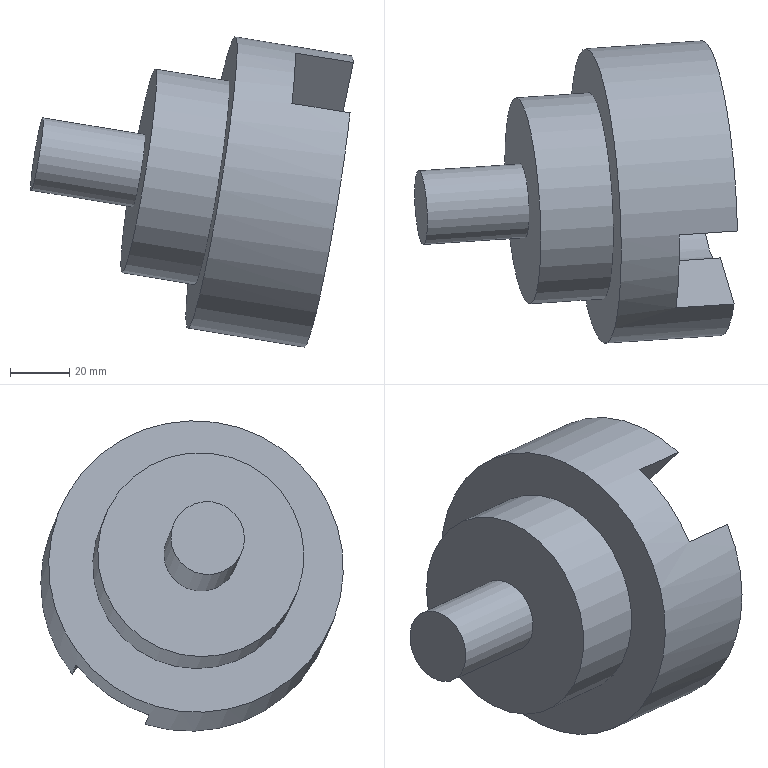Component | NX | 2 | 1 solid | 16 faces | volume 318011 mm3 | plane 12 | cylinder 4 | commonest cylinder face diameters 100 x1 50 x1 70 x1 25 x1